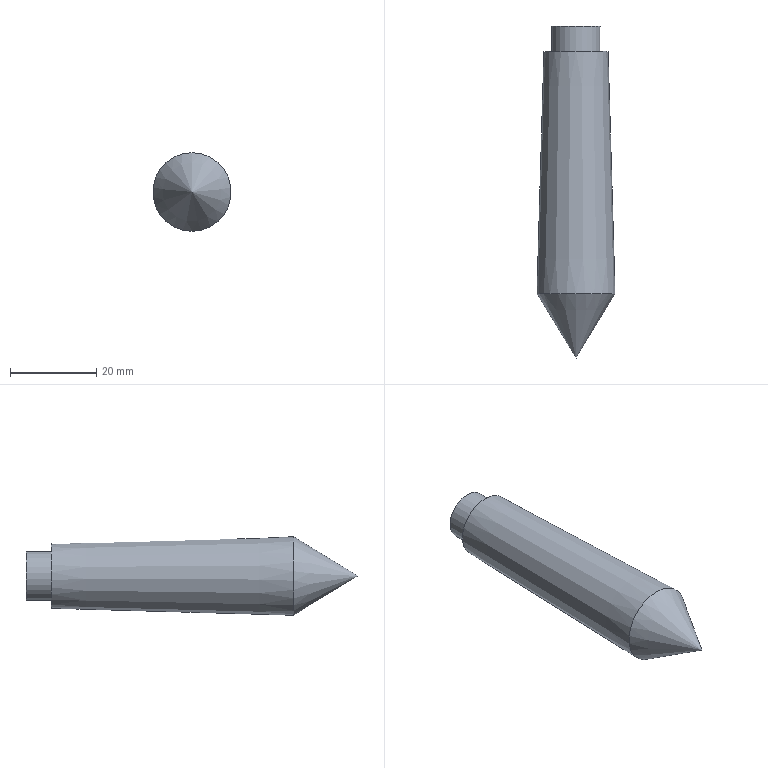Component | NX | LIVE_CENTER | 1 solid | 5 faces | box 18.23 x 77.06 x 18.23 mm | volume 14110 mm3 | cone 2 | plane 2 | cylinder 1 | commonest cylinder face diameters 11.299 x1
STEP:
#1=CARTESIAN_POINT('',(0.,0.,0.));
#2=DIRECTION('',(0.,0.,1.));
#3=DIRECTION('',(1.,0.,0.));
#4=AXIS2_PLACEMENT_3D('',#1,#2,#3);
#5=CARTESIAN_POINT('',(0.,-84.91,85.1));
#6=VERTEX_POINT('',#5);
#7=CARTESIAN_POINT('',(0.,-70.029,94.213));
#8=VERTEX_POINT('',#7);
#9=CARTESIAN_POINT('',(0.,-84.91,85.1));
#10=CARTESIAN_POINT('',(0.,-70.029,94.213));
#11=B_SPLINE_CURVE_WITH_KNOTS('',1,(#9,#10),.UNSPECIFIED.,.F.,.F.,(2,2),(-17.45,0.),.PIECEWISE_BEZIER_KNOTS.);
#12=CARTESIAN_POINT('',(0.,-70.029,85.1));
#13=DIRECTION('',(0.,1.,0.));
#14=DIRECTION('',(0.,0.,1.));
#15=AXIS2_PLACEMENT_3D('',#12,#13,#14);
#16=CONICAL_SURFACE('',#15,9.113,0.5495);
#17=CARTESIAN_POINT('',(6.283,0.));
#18=DIRECTION('',(0.,1.));
#19=VECTOR('',#18,1.);
#20=LINE('',#17,#19);
#21=(GEOMETRIC_REPRESENTATION_CONTEXT(2)PARAMETRIC_REPRESENTATION_CONTEXT()REPRESENTATION_CONTEXT('',''));
#22=DEFINITIONAL_REPRESENTATION('',(#20),#21);
#23=PCURVE('',#16,#22);
#24=CARTESIAN_POINT('',(0.,0.));
#25=DIRECTION('',(0.,1.));
#26=VECTOR('',#25,1.);
#27=LINE('',#24,#26);
#28=(GEOMETRIC_REPRESENTATION_CONTEXT(2)PARAMETRIC_REPRESENTATION_CONTEXT()REPRESENTATION_CONTEXT('',''));
#29=DEFINITIONAL_REPRESENTATION('',(#27),#28);
#30=PCURVE('',#16,#29);
#31=SEAM_CURVE('',#11,(#23,#30),.PCURVE_S1.);
#32=EDGE_CURVE('',#6,#8,#31,.T.);
#33=ORIENTED_EDGE('',*,*,#32,.T.);
#34=CARTESIAN_POINT('',(0.,-70.029,75.987));
#35=VERTEX_POINT('',#34);
#36=CARTESIAN_POINT('',(0.,-70.029,85.1));
#37=DIRECTION('',(0.,-1.,0.));
#38=DIRECTION('',(0.,0.,-1.));
#39=AXIS2_PLACEMENT_3D('',#36,#37,#38);
#40=CIRCLE('',#39,9.113);
#41=CARTESIAN_POINT('',(9.425,0.));
#42=DIRECTION('',(-1.,0.));
#43=VECTOR('',#42,1.);
#44=LINE('',#41,#43);
#45=(GEOMETRIC_REPRESENTATION_CONTEXT(2)PARAMETRIC_REPRESENTATION_CONTEXT()REPRESENTATION_CONTEXT('',''));
#46=DEFINITIONAL_REPRESENTATION('',(#44),#45);
#47=PCURVE('',#16,#46);
#48=CARTESIAN_POINT('',(0.,-13.763,85.1));
#49=DIRECTION('',(0.,-1.,0.));
#50=DIRECTION('',(0.,0.,-1.));
#51=AXIS2_PLACEMENT_3D('',#48,#49,#50);
#52=CONICAL_SURFACE('',#51,7.491,0.02882);
#53=CARTESIAN_POINT('',(0.,56.266));
#54=DIRECTION('',(1.,0.));
#55=VECTOR('',#54,1.);
#56=LINE('',#53,#55);
#57=(GEOMETRIC_REPRESENTATION_CONTEXT(2)PARAMETRIC_REPRESENTATION_CONTEXT()REPRESENTATION_CONTEXT('',''));
#58=DEFINITIONAL_REPRESENTATION('',(#56),#57);
#59=PCURVE('',#52,#58);
#60=SURFACE_CURVE('',#40,(#47,#59),.PCURVE_S1.);
#61=EDGE_CURVE('',#8,#35,#60,.T.);
#62=ORIENTED_EDGE('',*,*,#61,.T.);
#63=CARTESIAN_POINT('',(0.,-70.029,85.1));
#64=DIRECTION('',(0.,-1.,0.));
#65=DIRECTION('',(0.,0.,-1.));
#66=AXIS2_PLACEMENT_3D('',#63,#64,#65);
#67=CIRCLE('',#66,9.113);
#68=CARTESIAN_POINT('',(3.142,0.));
#69=DIRECTION('',(-1.,0.));
#70=VECTOR('',#69,1.);
#71=LINE('',#68,#70);
#72=(GEOMETRIC_REPRESENTATION_CONTEXT(2)PARAMETRIC_REPRESENTATION_CONTEXT()REPRESENTATION_CONTEXT('',''));
#73=DEFINITIONAL_REPRESENTATION('',(#71),#72);
#74=PCURVE('',#16,#73);
#75=CARTESIAN_POINT('',(0.,56.266));
#76=DIRECTION('',(1.,0.));
#77=VECTOR('',#76,1.);
#78=LINE('',#75,#77);
#79=(GEOMETRIC_REPRESENTATION_CONTEXT(2)PARAMETRIC_REPRESENTATION_CONTEXT()REPRESENTATION_CONTEXT('',''));
#80=DEFINITIONAL_REPRESENTATION('',(#78),#79);
#81=PCURVE('',#52,#80);
#82=SURFACE_CURVE('',#67,(#74,#81),.PCURVE_S1.);
#83=EDGE_CURVE('',#35,#8,#82,.T.);
#84=ORIENTED_EDGE('',*,*,#83,.T.);
#85=ORIENTED_EDGE('',*,*,#32,.F.);
#86=EDGE_LOOP('',(#33,#62,#84,#85));
#87=FACE_BOUND('',#86,.T.);
#88=ADVANCED_FACE('',(#87),#16,.T.);
#89=CARTESIAN_POINT('',(0.,-7.849,79.45));
#90=VERTEX_POINT('',#89);
#91=CARTESIAN_POINT('',(0.,-7.849,85.1));
#92=DIRECTION('',(0.,-1.,0.));
#93=DIRECTION('',(0.,0.,-1.));
#94=AXIS2_PLACEMENT_3D('',#91,#92,#93);
#95=CIRCLE('',#94,5.65);
#96=CARTESIAN_POINT('',(0.,-7.849,85.1));
#97=DIRECTION('',(0.,-1.,0.));
#98=DIRECTION('',(0.,0.,-1.));
#99=AXIS2_PLACEMENT_3D('',#96,#97,#98);
#100=PLANE('',#99);
#101=CARTESIAN_POINT('',(0.,0.));
#102=DIRECTION('',(1.,0.));
#103=AXIS2_PLACEMENT_2D('',#101,#102);
#104=CIRCLE('',#103,5.65);
#105=(GEOMETRIC_REPRESENTATION_CONTEXT(2)PARAMETRIC_REPRESENTATION_CONTEXT()REPRESENTATION_CONTEXT('',''));
#106=DEFINITIONAL_REPRESENTATION('',(#104),#105);
#107=PCURVE('',#100,#106);
#108=CARTESIAN_POINT('',(0.,-7.849,85.1));
#109=DIRECTION('',(0.,-1.,0.));
#110=DIRECTION('',(0.,0.,-1.));
#111=AXIS2_PLACEMENT_3D('',#108,#109,#110);
#112=CYLINDRICAL_SURFACE('',#111,5.65);
#113=CARTESIAN_POINT('',(0.,0.));
#114=DIRECTION('',(1.,0.));
#115=VECTOR('',#114,1.);
#116=LINE('',#113,#115);
#117=(GEOMETRIC_REPRESENTATION_CONTEXT(2)PARAMETRIC_REPRESENTATION_CONTEXT()REPRESENTATION_CONTEXT('',''));
#118=DEFINITIONAL_REPRESENTATION('',(#116),#117);
#119=PCURVE('',#112,#118);
#120=SURFACE_CURVE('',#95,(#107,#119),.PCURVE_S1.);
#121=EDGE_CURVE('',#90,#90,#120,.T.);
#122=ORIENTED_EDGE('',*,*,#121,.F.);
#123=EDGE_LOOP('',(#122));
#124=FACE_BOUND('',#123,.T.);
#125=ADVANCED_FACE('',(#124),#100,.F.);
#126=CARTESIAN_POINT('',(0.,-13.763,79.45));
#127=VERTEX_POINT('',#126);
#128=CARTESIAN_POINT('',(0.,-13.763,85.1));
#129=DIRECTION('',(0.,-1.,0.));
#130=DIRECTION('',(0.,0.,-1.));
#131=AXIS2_PLACEMENT_3D('',#128,#129,#130);
#132=CIRCLE('',#131,5.65);
#133=CARTESIAN_POINT('',(0.,5.914));
#134=DIRECTION('',(1.,0.));
#135=VECTOR('',#134,1.);
#136=LINE('',#133,#135);
#137=(GEOMETRIC_REPRESENTATION_CONTEXT(2)PARAMETRIC_REPRESENTATION_CONTEXT()REPRESENTATION_CONTEXT('',''));
#138=DEFINITIONAL_REPRESENTATION('',(#136),#137);
#139=PCURVE('',#112,#138);
#140=CARTESIAN_POINT('',(0.,-13.763,90.75));
#141=DIRECTION('',(0.,-1.,0.));
#142=DIRECTION('',(0.,0.,-1.));
#143=AXIS2_PLACEMENT_3D('',#140,#141,#142);
#144=PLANE('',#143);
#145=CARTESIAN_POINT('',(5.65,0.));
#146=DIRECTION('',(1.,0.));
#147=AXIS2_PLACEMENT_2D('',#145,#146);
#148=CIRCLE('',#147,5.65);
#149=(GEOMETRIC_REPRESENTATION_CONTEXT(2)PARAMETRIC_REPRESENTATION_CONTEXT()REPRESENTATION_CONTEXT('',''));
#150=DEFINITIONAL_REPRESENTATION('',(#148),#149);
#151=PCURVE('',#144,#150);
#152=SURFACE_CURVE('',#132,(#139,#151),.PCURVE_S1.);
#153=EDGE_CURVE('',#127,#127,#152,.T.);
#154=ORIENTED_EDGE('',*,*,#153,.F.);
#155=CARTESIAN_POINT('',(-0.,-7.849,79.45));
#156=CARTESIAN_POINT('',(-0.,-13.763,79.45));
#157=B_SPLINE_CURVE_WITH_KNOTS('',1,(#155,#156),.UNSPECIFIED.,.F.,.F.,(2,2),(0.,5.914),.PIECEWISE_BEZIER_KNOTS.);
#158=CARTESIAN_POINT('',(0.,0.));
#159=DIRECTION('',(0.,1.));
#160=VECTOR('',#159,1.);
#161=LINE('',#158,#160);
#162=(GEOMETRIC_REPRESENTATION_CONTEXT(2)PARAMETRIC_REPRESENTATION_CONTEXT()REPRESENTATION_CONTEXT('',''));
#163=DEFINITIONAL_REPRESENTATION('',(#161),#162);
#164=PCURVE('',#112,#163);
#165=CARTESIAN_POINT('',(6.283,0.));
#166=DIRECTION('',(0.,1.));
#167=VECTOR('',#166,1.);
#168=LINE('',#165,#167);
#169=(GEOMETRIC_REPRESENTATION_CONTEXT(2)PARAMETRIC_REPRESENTATION_CONTEXT()REPRESENTATION_CONTEXT('',''));
#170=DEFINITIONAL_REPRESENTATION('',(#168),#169);
#171=PCURVE('',#112,#170);
#172=SEAM_CURVE('',#157,(#164,#171),.PCURVE_S1.);
#173=EDGE_CURVE('',#90,#127,#172,.T.);
#174=ORIENTED_EDGE('',*,*,#173,.F.);
#175=ORIENTED_EDGE('',*,*,#121,.T.);
#176=ORIENTED_EDGE('',*,*,#173,.T.);
#177=EDGE_LOOP('',(#154,#174,#175,#176));
#178=FACE_BOUND('',#177,.T.);
#179=ADVANCED_FACE('',(#178),#112,.T.);
#180=CARTESIAN_POINT('',(0.,-13.763,77.609));
#181=VERTEX_POINT('',#180);
#182=CARTESIAN_POINT('',(0.,-13.763,85.1));
#183=DIRECTION('',(0.,-1.,0.));
#184=DIRECTION('',(0.,0.,-1.));
#185=AXIS2_PLACEMENT_3D('',#182,#183,#184);
#186=CIRCLE('',#185,7.491);
#187=CARTESIAN_POINT('',(5.65,0.));
#188=DIRECTION('',(1.,0.));
#189=AXIS2_PLACEMENT_2D('',#187,#188);
#190=CIRCLE('',#189,7.491);
#191=(GEOMETRIC_REPRESENTATION_CONTEXT(2)PARAMETRIC_REPRESENTATION_CONTEXT()REPRESENTATION_CONTEXT('',''));
#192=DEFINITIONAL_REPRESENTATION('',(#190),#191);
#193=PCURVE('',#144,#192);
#194=CARTESIAN_POINT('',(0.,-0.));
#195=DIRECTION('',(1.,0.));
#196=VECTOR('',#195,1.);
#197=LINE('',#194,#196);
#198=(GEOMETRIC_REPRESENTATION_CONTEXT(2)PARAMETRIC_REPRESENTATION_CONTEXT()REPRESENTATION_CONTEXT('',''));
#199=DEFINITIONAL_REPRESENTATION('',(#197),#198);
#200=PCURVE('',#52,#199);
#201=SURFACE_CURVE('',#186,(#193,#200),.PCURVE_S1.);
#202=EDGE_CURVE('',#181,#181,#201,.T.);
#203=ORIENTED_EDGE('',*,*,#202,.F.);
#204=EDGE_LOOP('',(#203));
#205=FACE_BOUND('',#204,.T.);
#206=ORIENTED_EDGE('',*,*,#153,.T.);
#207=EDGE_LOOP('',(#206));
#208=FACE_BOUND('',#207,.T.);
#209=ADVANCED_FACE('',(#205,#208),#144,.F.);
#210=ORIENTED_EDGE('',*,*,#83,.F.);
#211=CARTESIAN_POINT('',(-0.,-13.763,77.609));
#212=CARTESIAN_POINT('',(-0.,-70.029,75.987));
#213=B_SPLINE_CURVE_WITH_KNOTS('',1,(#211,#212),.UNSPECIFIED.,.F.,.F.,(2,2),(-0.,56.289),.PIECEWISE_BEZIER_KNOTS.);
#214=CARTESIAN_POINT('',(0.,0.));
#215=DIRECTION('',(0.,1.));
#216=VECTOR('',#215,1.);
#217=LINE('',#214,#216);
#218=(GEOMETRIC_REPRESENTATION_CONTEXT(2)PARAMETRIC_REPRESENTATION_CONTEXT()REPRESENTATION_CONTEXT('',''));
#219=DEFINITIONAL_REPRESENTATION('',(#217),#218);
#220=PCURVE('',#52,#219);
#221=CARTESIAN_POINT('',(6.283,0.));
#222=DIRECTION('',(0.,1.));
#223=VECTOR('',#222,1.);
#224=LINE('',#221,#223);
#225=(GEOMETRIC_REPRESENTATION_CONTEXT(2)PARAMETRIC_REPRESENTATION_CONTEXT()REPRESENTATION_CONTEXT('',''));
#226=DEFINITIONAL_REPRESENTATION('',(#224),#225);
#227=PCURVE('',#52,#226);
#228=SEAM_CURVE('',#213,(#220,#227),.PCURVE_S1.);
#229=EDGE_CURVE('',#181,#35,#228,.T.);
#230=ORIENTED_EDGE('',*,*,#229,.F.);
#231=ORIENTED_EDGE('',*,*,#202,.T.);
#232=ORIENTED_EDGE('',*,*,#229,.T.);
#233=ORIENTED_EDGE('',*,*,#61,.F.);
#234=EDGE_LOOP('',(#210,#230,#231,#232,#233));
#235=FACE_BOUND('',#234,.T.);
#236=ADVANCED_FACE('',(#235),#52,.T.);
#237=CLOSED_SHELL('',(#88,#125,#179,#209,#236));
#238=MANIFOLD_SOLID_BREP('',#237);
#239=(LENGTH_UNIT()NAMED_UNIT(*)SI_UNIT(.MILLI.,.METRE.));
#240=UNCERTAINTY_MEASURE_WITH_UNIT(LENGTH_MEASURE(0.00001),#239,'','');
#241=(NAMED_UNIT(*)PLANE_ANGLE_UNIT()SI_UNIT($,.RADIAN.));
#242=(NAMED_UNIT(*)SI_UNIT($,.STERADIAN.)SOLID_ANGLE_UNIT());
#243=(GEOMETRIC_REPRESENTATION_CONTEXT(3)GLOBAL_UNCERTAINTY_ASSIGNED_CONTEXT((#240))GLOBAL_UNIT_ASSIGNED_CONTEXT((#239,#241,#242))REPRESENTATION_CONTEXT('',''));
#244=ADVANCED_BREP_SHAPE_REPRESENTATION('',(#4,#238),#243);